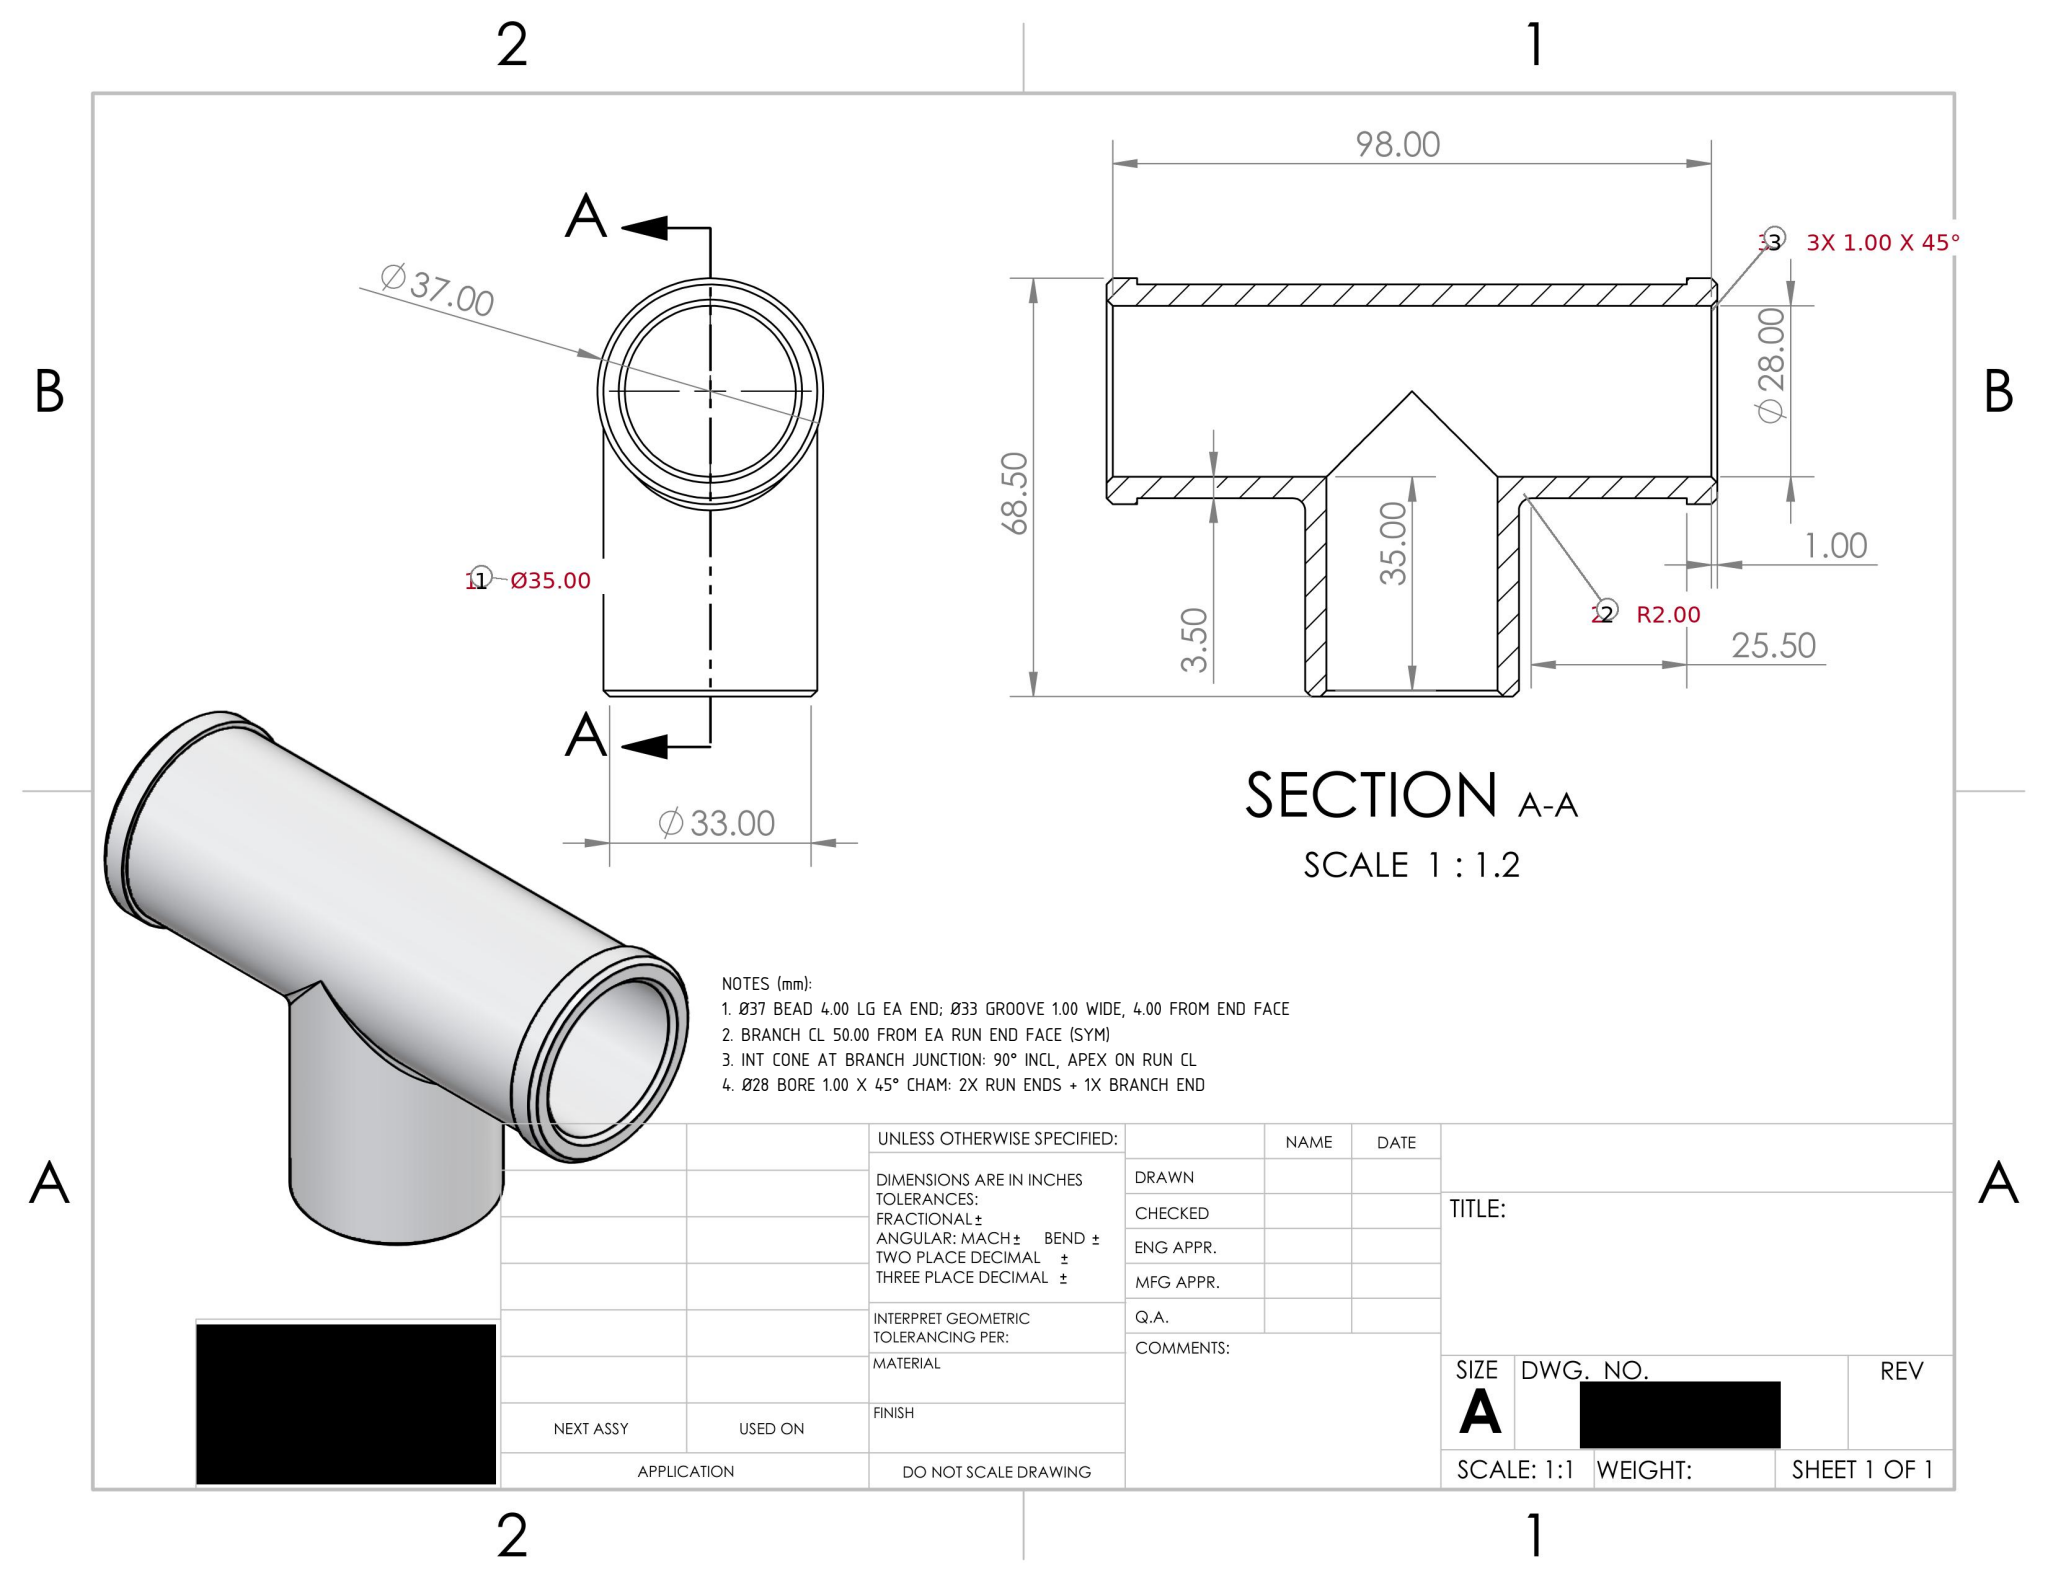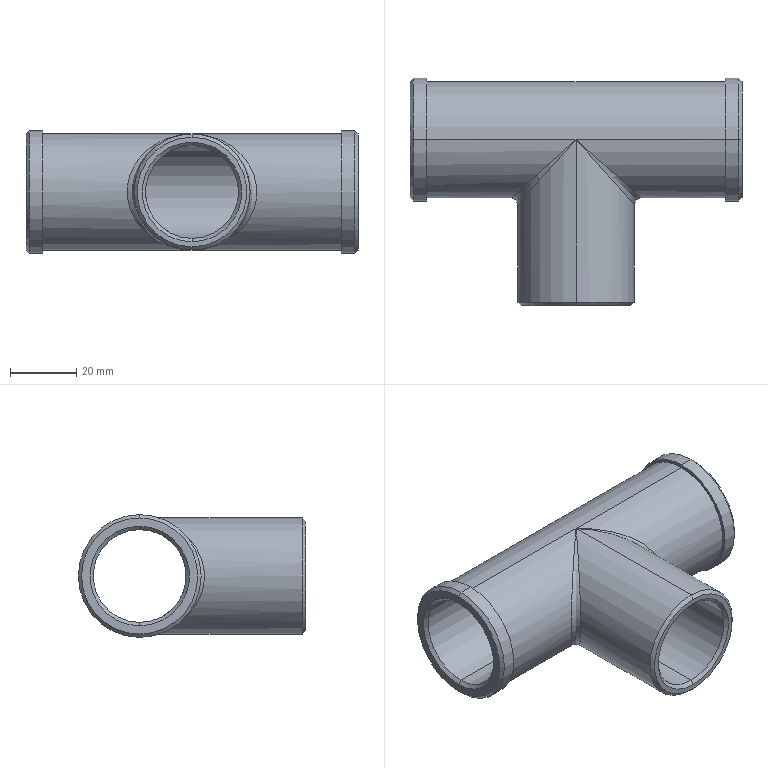Part | SolidWorks | mm | 1 solid | 33 faces | box 100 x 68.5 x 37 mm | volume 45845 mm3 | cylinder 14 | cone 12 | plane 5 | spline 2 | commonest cylinder face diameters 28 x5 35 x5 37 x4
Drawing notes:
Ø37 BEAD 4.00 LG EA END; Ø33 GROOVE 1.00 WIDE, 4.00 FROM END FACE | from the solid: Ø37 x-axis cyl length 4.00 at each run end; planes x=0/5 and x=95/100 bound bead+groove (groove inner face 5.00 from end face)
BRANCH CL 50.00 FROM EA RUN END FACE (SYM) | from the solid: y-axis (branch) cylinders Ø28/Ø35 at x=50.0; run end planes x=0 and x=100
INT CONE AT BRANCH JUNCTION: 90° INCL, APEX ON RUN CL | from the solid: cone included angle 90°, ref dia 28 (branch bore); run axis at y=50 / z=18.5, branch bore Ø28 on same CL
Ø28 BORE 1.00 X 45° CHAM: 2X RUN ENDS + 1X BRANCH END | from the solid: cones 90° incl ref dia 30 at Ø28 bore ends (run x=0, x=100 and branch y=0)